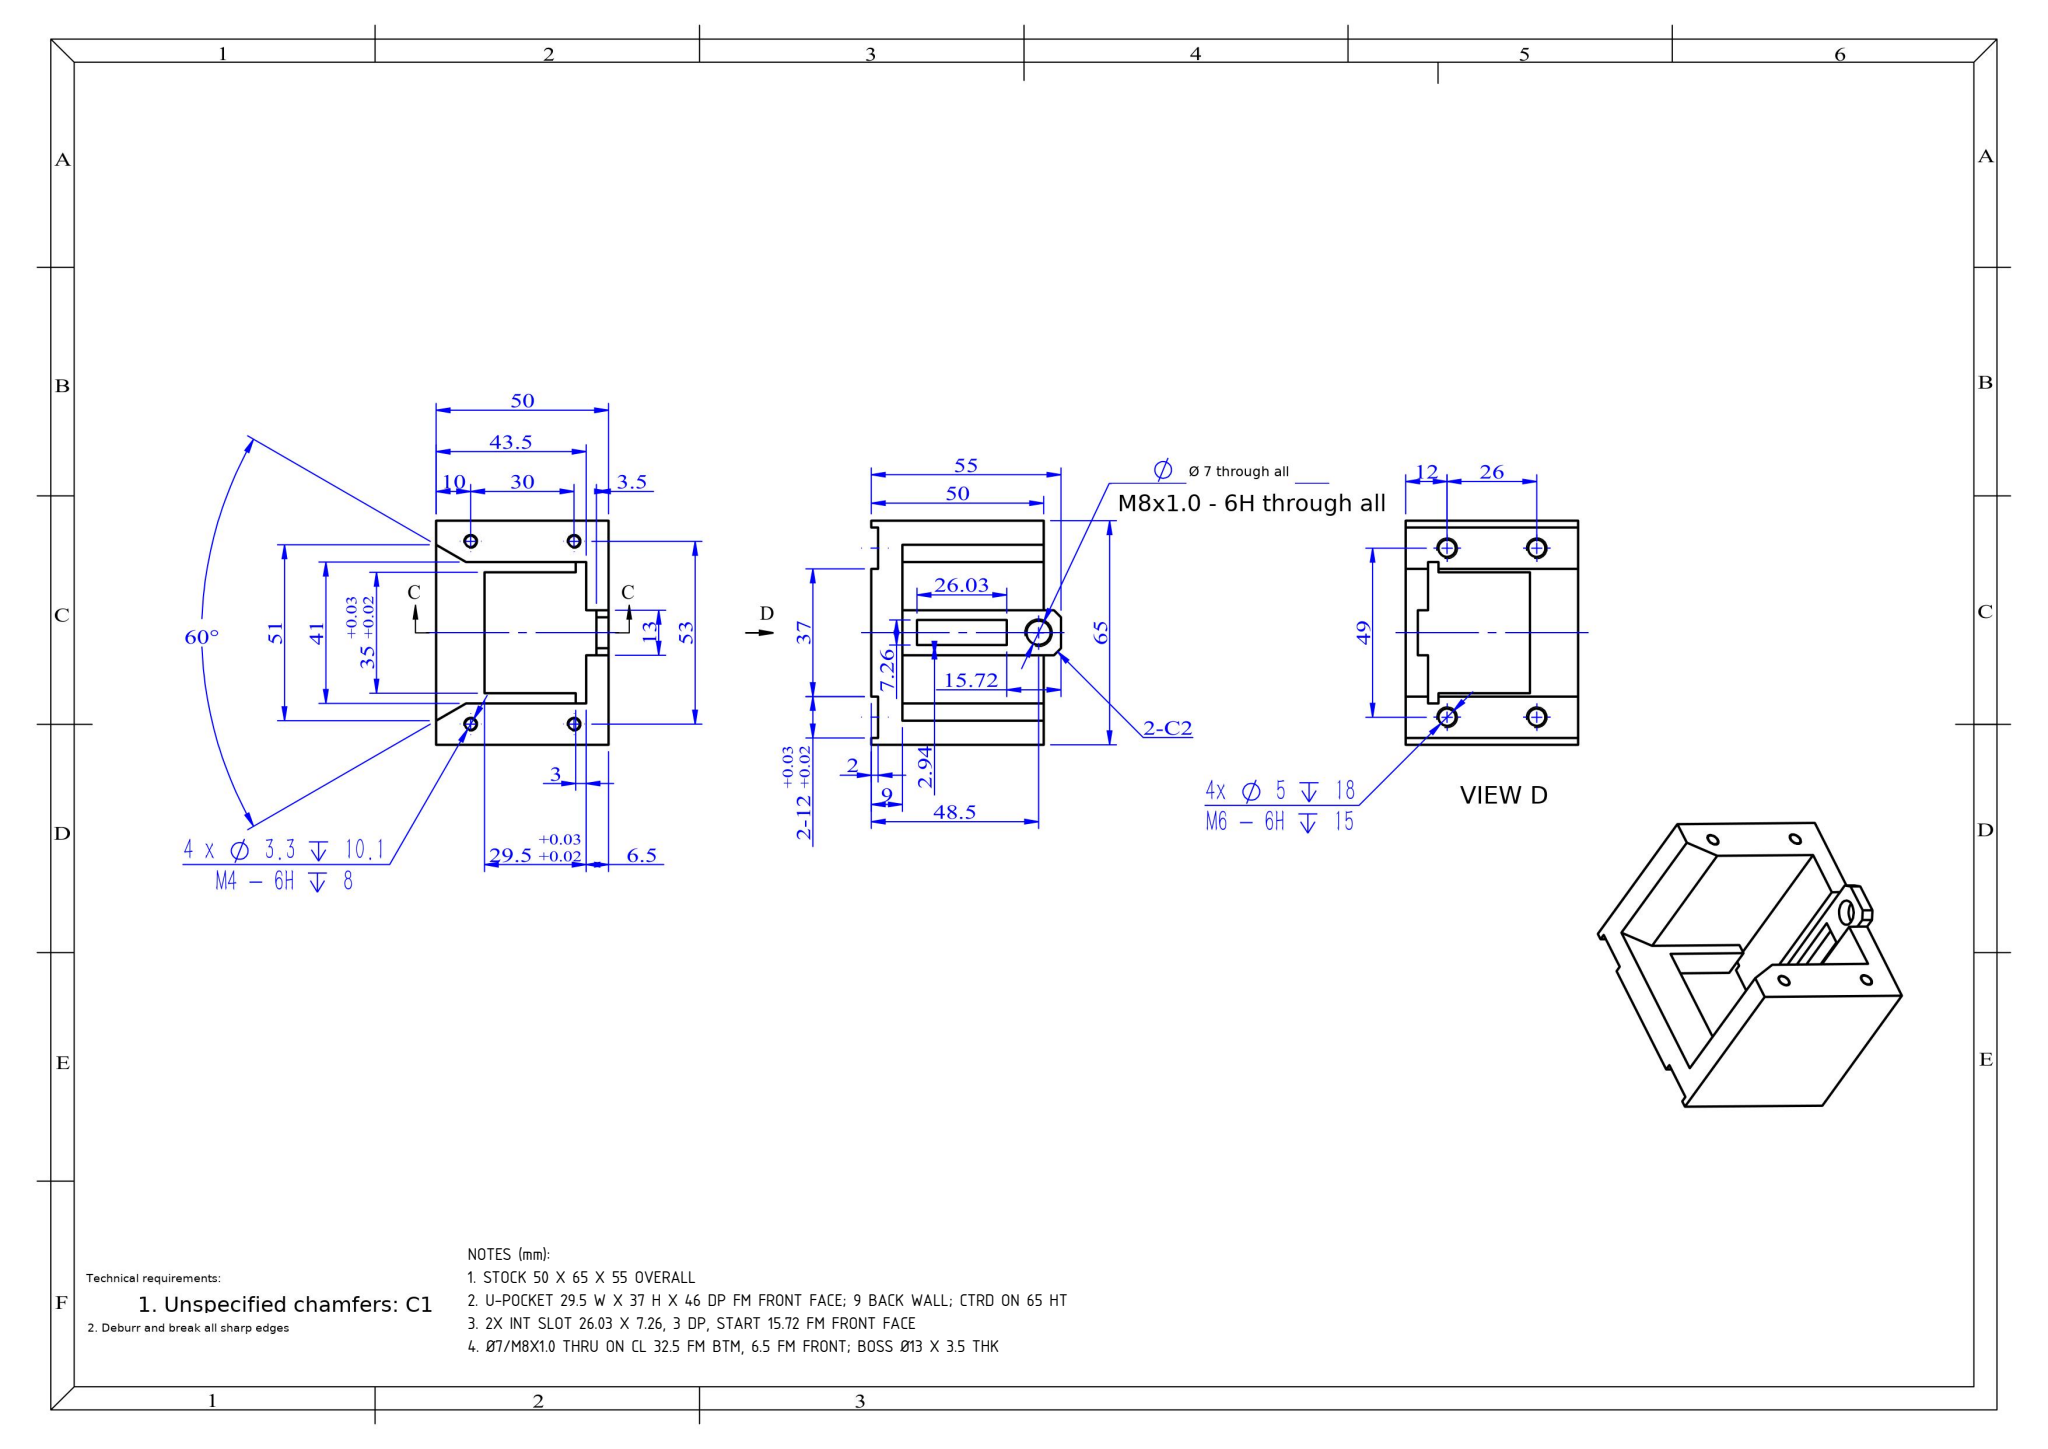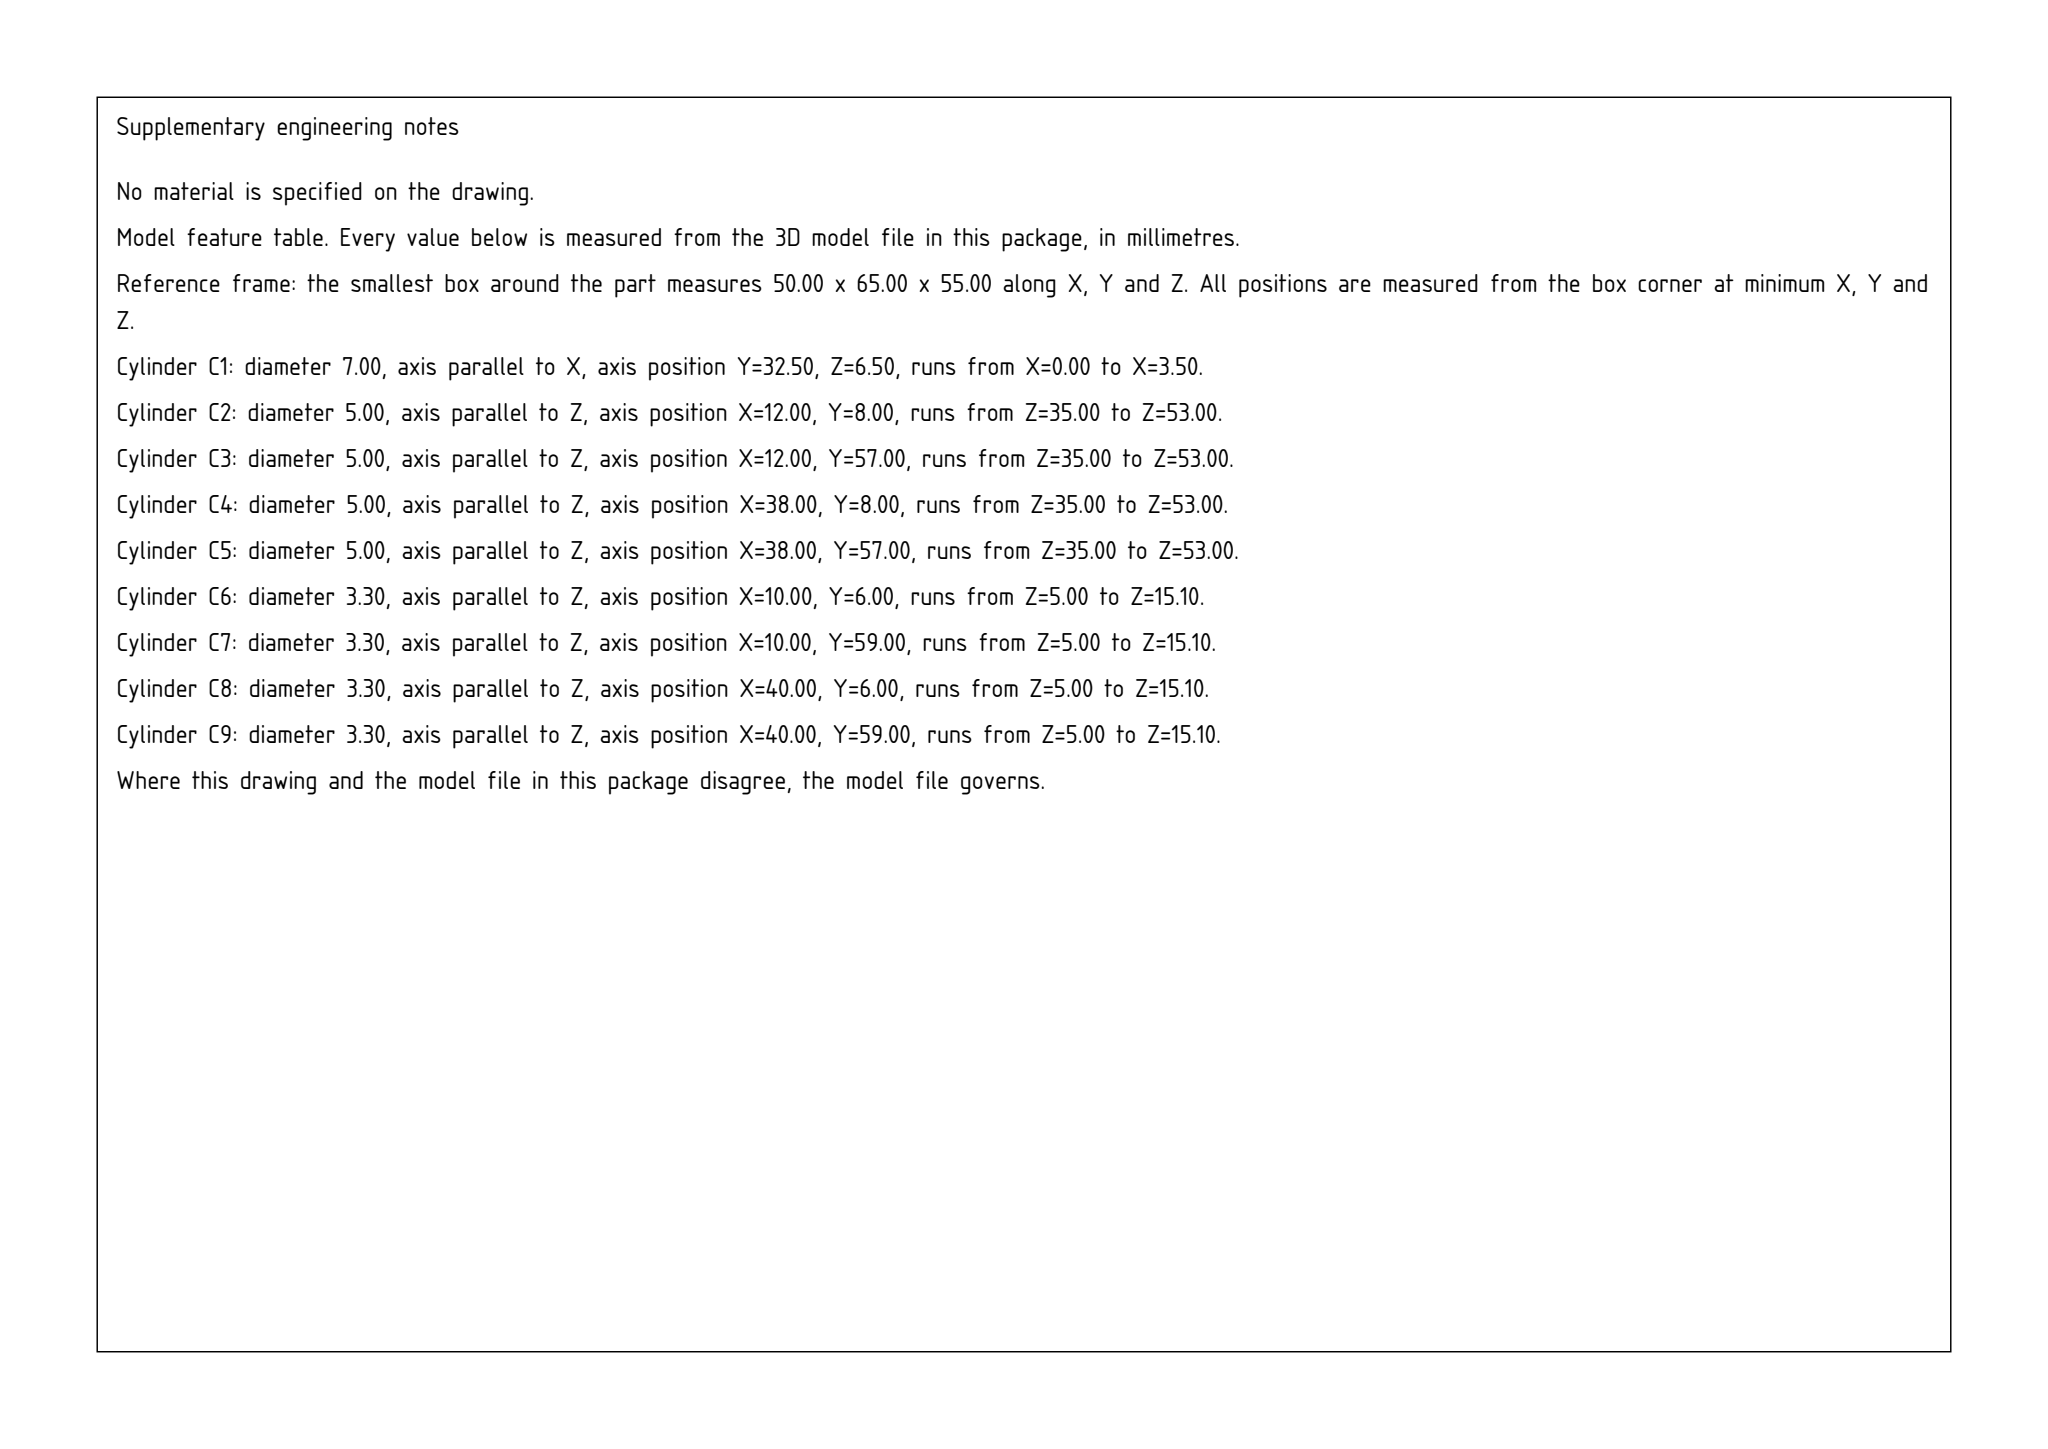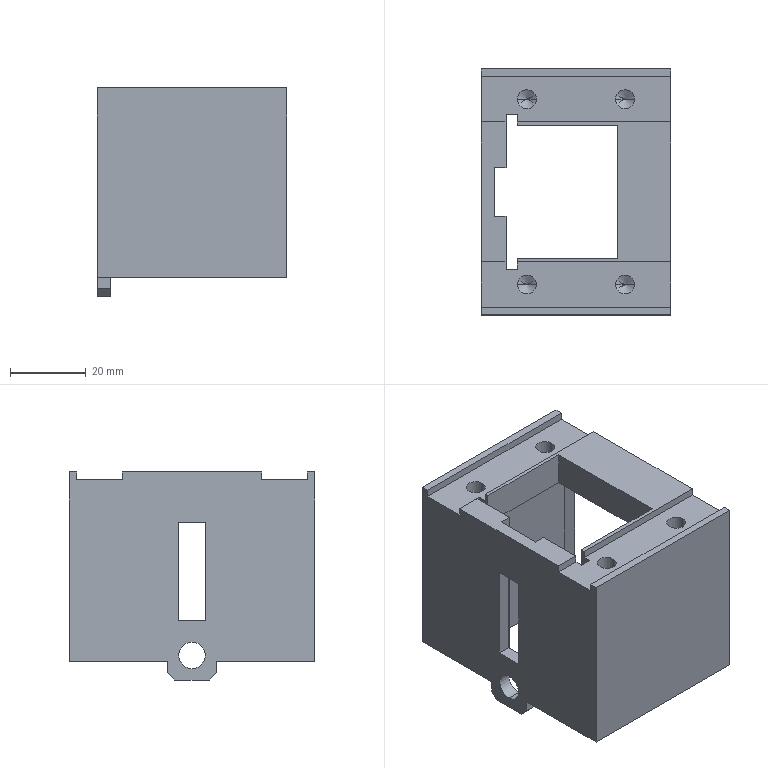Part | SolidWorks | mm | 1 solid | 76 faces | box 50 x 65 x 55 mm | volume 71429 mm3 | plane 42 | cylinder 18 | cone 16 | commonest cylinder face diameters 3.3 x8 5 x8 7 x2
Drawing notes:
STOCK 50 X 65 X 55 OVERALL | from the solid: bbox_xyz 50.0 x 65.0 x 55.0
U-POCKET 29.5 W X 37 H X 46 DP FM FRONT FACE; 9 BACK WALL; CTRD ON 65 HT | from the solid: x planes 6.5 & 36.0 = 29.5; y 14.0 & 51.0 = 37, sym abt 32.5 = 65/2; z floor 46.0, 55-46 = 9
2X INT SLOT 26.03 X 7.26, 3 DP, START 15.72 FM FRONT FACE | from the solid: z 15.72 to 41.74 = 26.02; y 28.94 to 36.19 = 7.25; x 6.5 to 9.5 = 3 dp
Ø7/M8X1.0 THRU ON CL 32.5 FM BTM, 6.5 FM FRONT; BOSS Ø13 X 3.5 THK | from the solid: cyl Ø7 axis x at y=32.5, z=6.5, len 3.5 (x 0-3.5); boss faces y=26 & y=39 give Ø13
build123d program:
from build123d import *

# Parameters (mm, degrees)
SKETCH1_W                  = 50
SKETCH1_H                  = 65
BOSS_EXTRUDE1_DEPTH        = 50
SKETCH2_W                  = 41
SKETCH2_H                  = 41
CUT_EXTRUDE1_DEPTH         = 43.5
SKETCH3_W                  = 29.5
SKETCH3_H                  = 35
CUT_EXTRUDE2_DEPTH         = 108.685
CHAMFER1_SIZE              = 5
CHAMFER1_SIZE2             = 8.66
SKETCH4_W                  = 6.5
SKETCH4_H                  = 13
BOSS_EXTRUDE2_DEPTH        = 5
M8X1_0_TAPPED_HOLE1_D      = 7
CHAMFER2_SIZE              = 2
SKETCH15_W                 = 2
SKETCH15_H                 = 12
CUT_EXTRUDE5_DEPTH         = 86.162
M6_TAPPED_HOLE1_AT_2_COUNT = 2
M6_TAPPED_HOLE1_AT_2_PITCH = 26
SKETCH20_W                 = 3
SKETCH20_H                 = 3
CUT_EXTRUDE6_DEPTH         = 106.887
SKETCH22_W                 = 3
SKETCH22_H                 = 13
CUT_EXTRUDE8_DEPTH         = 111.096
M4_TAPPED_HOLE1_AT_2_COUNT = 2
M4_TAPPED_HOLE1_AT_2_PITCH = 30
SKETCH25_W                 = 26.025
SKETCH25_H                 = 7.255
CUT_EXTRUDE9_DEPTH         = 10


with BuildPart() as part:
    # Sketch1 → Boss-Extrude1 (new body)
    with BuildSketch(Plane.XY):
        with Locations((57.726, 14.96)):
            Rectangle(SKETCH1_W, SKETCH1_H)
    extrude(amount=BOSS_EXTRUDE1_DEPTH)

    # Sketch2 → Cut-Extrude1 (cut)
    with BuildSketch(Plane(origin=(82.726, 0, 0), x_dir=(0, 0, -1), z_dir=(1, 0, 0))):
        with Locations((-20.5, 14.96)):
            Rectangle(SKETCH2_W, SKETCH2_H)
    extrude(amount=-CUT_EXTRUDE1_DEPTH, mode=Mode.SUBTRACT)

    # Sketch3 → Cut-Extrude2 (cut, through all)
    with BuildSketch(Plane.XY.offset(50)):
        with Locations((53.976, 14.96)):
            Rectangle(SKETCH3_W, SKETCH3_H)
    extrude(amount=-CUT_EXTRUDE2_DEPTH, mode=Mode.SUBTRACT)

    # Chamfer1
    chamfer1_edges = [part.edges().sort_by_distance(p)[0] for p in [
        (82.726, 35.46, 20.5),
        (82.726, -5.54, 20.5),
    ]]
    chamfer1_side = [part.faces().sort_by_distance(p)[0] for p in [
        (82.726, -11.54, 0.8201),
    ]]
    chamfer(chamfer1_edges, length=CHAMFER1_SIZE, length2=CHAMFER1_SIZE2, reference=chamfer1_side[0])

    # Sketch4 → Boss-Extrude2 (add)
    with BuildSketch(Plane(origin=(0, 0, 0), x_dir=(-1, 0, 0), z_dir=(0, 0, -1))):
        with Locations((-35.976, 14.96)):
            Rectangle(SKETCH4_W, SKETCH4_H)
    extrude(amount=BOSS_EXTRUDE2_DEPTH)

    # M8x1.0 Tapped Hole1 (through all)
    with Locations(Plane.ZY.offset(-32.726)):
        with Locations((1.5, 14.96)):
            Hole(M8X1_0_TAPPED_HOLE1_D / 2)

    # Chamfer2
    chamfer2_edges = [part.edges().sort_by_distance(p)[0] for p in [
        (35.976, 8.46, -5),
        (35.976, 21.46, -5),
    ]]
    chamfer(chamfer2_edges, length=CHAMFER2_SIZE)

    # Sketch15 → Cut-Extrude5 (cut, through all)
    with BuildSketch(Plane.ZY.offset(-32.726)):
        with Locations((49, -9.54)):
            Rectangle(SKETCH15_W, SKETCH15_H)
    cut_extrude5 = extrude(amount=-CUT_EXTRUDE5_DEPTH, mode=Mode.SUBTRACT)

    # Mirror2: Cut-Extrude5 across plane
    add(cut_extrude5.mirror(Plane.ZX.offset(14.96)), mode=Mode.SUBTRACT)

    # Sketch17 → M6 Tapped Hole1 (revolve, cut)
    with BuildSketch(Plane(origin=(70.726, -9.54, 48), x_dir=(0, -1, 0), z_dir=(1, 0, 0))):
        Polygon((0, 0), (0, 19.502), (2.5, 18), (2.5, 0), align=None)
    m6_tapped_hole1 = revolve(axis=Axis((70.726, -9.54, 54.35), (0, 0, -1)), mode=Mode.SUBTRACT)

    # M6 Tapped Hole1 at 2: M6 Tapped Hole1 ×2
    with Locations(*[(-i * M6_TAPPED_HOLE1_AT_2_PITCH, 0, 0) for i in range(1, M6_TAPPED_HOLE1_AT_2_COUNT)]):
        add(m6_tapped_hole1, mode=Mode.SUBTRACT)

    # Mirror3: M6 Tapped Hole1 across plane
    add(m6_tapped_hole1.mirror(Plane.ZX.offset(14.96)), mode=Mode.SUBTRACT)

    # Mirror3 copy 1 sketch → Mirror3 copy 1 (revolve, cut)
    with BuildSketch(Plane(origin=(44.726, 39.46, 48), x_dir=(0, 1, 0), z_dir=(1, 0, 0))):
        Polygon((0, 0), (0, -19.502), (2.5, -18), (2.5, 0), align=None)
    revolve(axis=Axis((44.726, 39.46, 54.35), (0, 0, 1)), mode=Mode.SUBTRACT)

    # Sketch20 → Cut-Extrude6 (cut, through all)
    with BuildSketch(Plane(origin=(0, 0, 41), x_dir=(-1, 0, 0), z_dir=(0, 0, -1))):
        with Locations((-40.726, 33.96)):
            Rectangle(SKETCH20_W, SKETCH20_H)
        with Locations((-40.726, -4.04)):
            Rectangle(SKETCH20_W, SKETCH20_H)
    extrude(amount=-CUT_EXTRUDE6_DEPTH, mode=Mode.SUBTRACT)

    # Sketch22 → Cut-Extrude8 (cut, through all)
    with BuildSketch(Plane(origin=(0, 0, -5), x_dir=(-1, 0, 0), z_dir=(0, 0, -1))):
        with Locations((-37.726, 14.96)):
            Rectangle(SKETCH22_W, SKETCH22_H)
    extrude(amount=-CUT_EXTRUDE8_DEPTH, mode=Mode.SUBTRACT)

    # Sketch24 → M4 Tapped Hole1 (revolve, cut)
    with BuildSketch(Plane(origin=(72.726, -11.54, 0), x_dir=(0, 1, 0), z_dir=(1, 0, 0))):
        Polygon((0, 0), (0, 11.091), (1.65, 10.1), (1.65, 0), align=None)
    m4_tapped_hole1 = revolve(axis=Axis((72.726, -11.54, -6.35), (0, 0, 1)), mode=Mode.SUBTRACT)

    # M4 Tapped Hole1 at 2: M4 Tapped Hole1 ×2
    with Locations(*[(-i * M4_TAPPED_HOLE1_AT_2_PITCH, 0, 0) for i in range(1, M4_TAPPED_HOLE1_AT_2_COUNT)]):
        add(m4_tapped_hole1, mode=Mode.SUBTRACT)

    # Mirror4: M4 Tapped Hole1 across plane
    add(m4_tapped_hole1.mirror(Plane.ZX.offset(14.96)), mode=Mode.SUBTRACT)

    # Mirror4 copy 1 sketch → Mirror4 copy 1 (revolve, cut)
    with BuildSketch(Plane(origin=(42.726, 41.46, 0), x_dir=(0, -1, 0), z_dir=(1, 0, 0))):
        Polygon((0, 0), (0, -11.091), (1.65, -10.1), (1.65, 0), align=None)
    revolve(axis=Axis((42.726, 41.46, -6.35), (0, 0, -1)), mode=Mode.SUBTRACT)

    # Sketch25 → Cut-Extrude9 (cut)
    with BuildSketch(Plane(origin=(36.226, 0, 0), x_dir=(0, 0, -1), z_dir=(1, 0, 0))):
        with Locations((-23.731, 15.027)):
            Rectangle(SKETCH25_W, SKETCH25_H)
    extrude(amount=-CUT_EXTRUDE9_DEPTH, mode=Mode.SUBTRACT)


solid = part.part